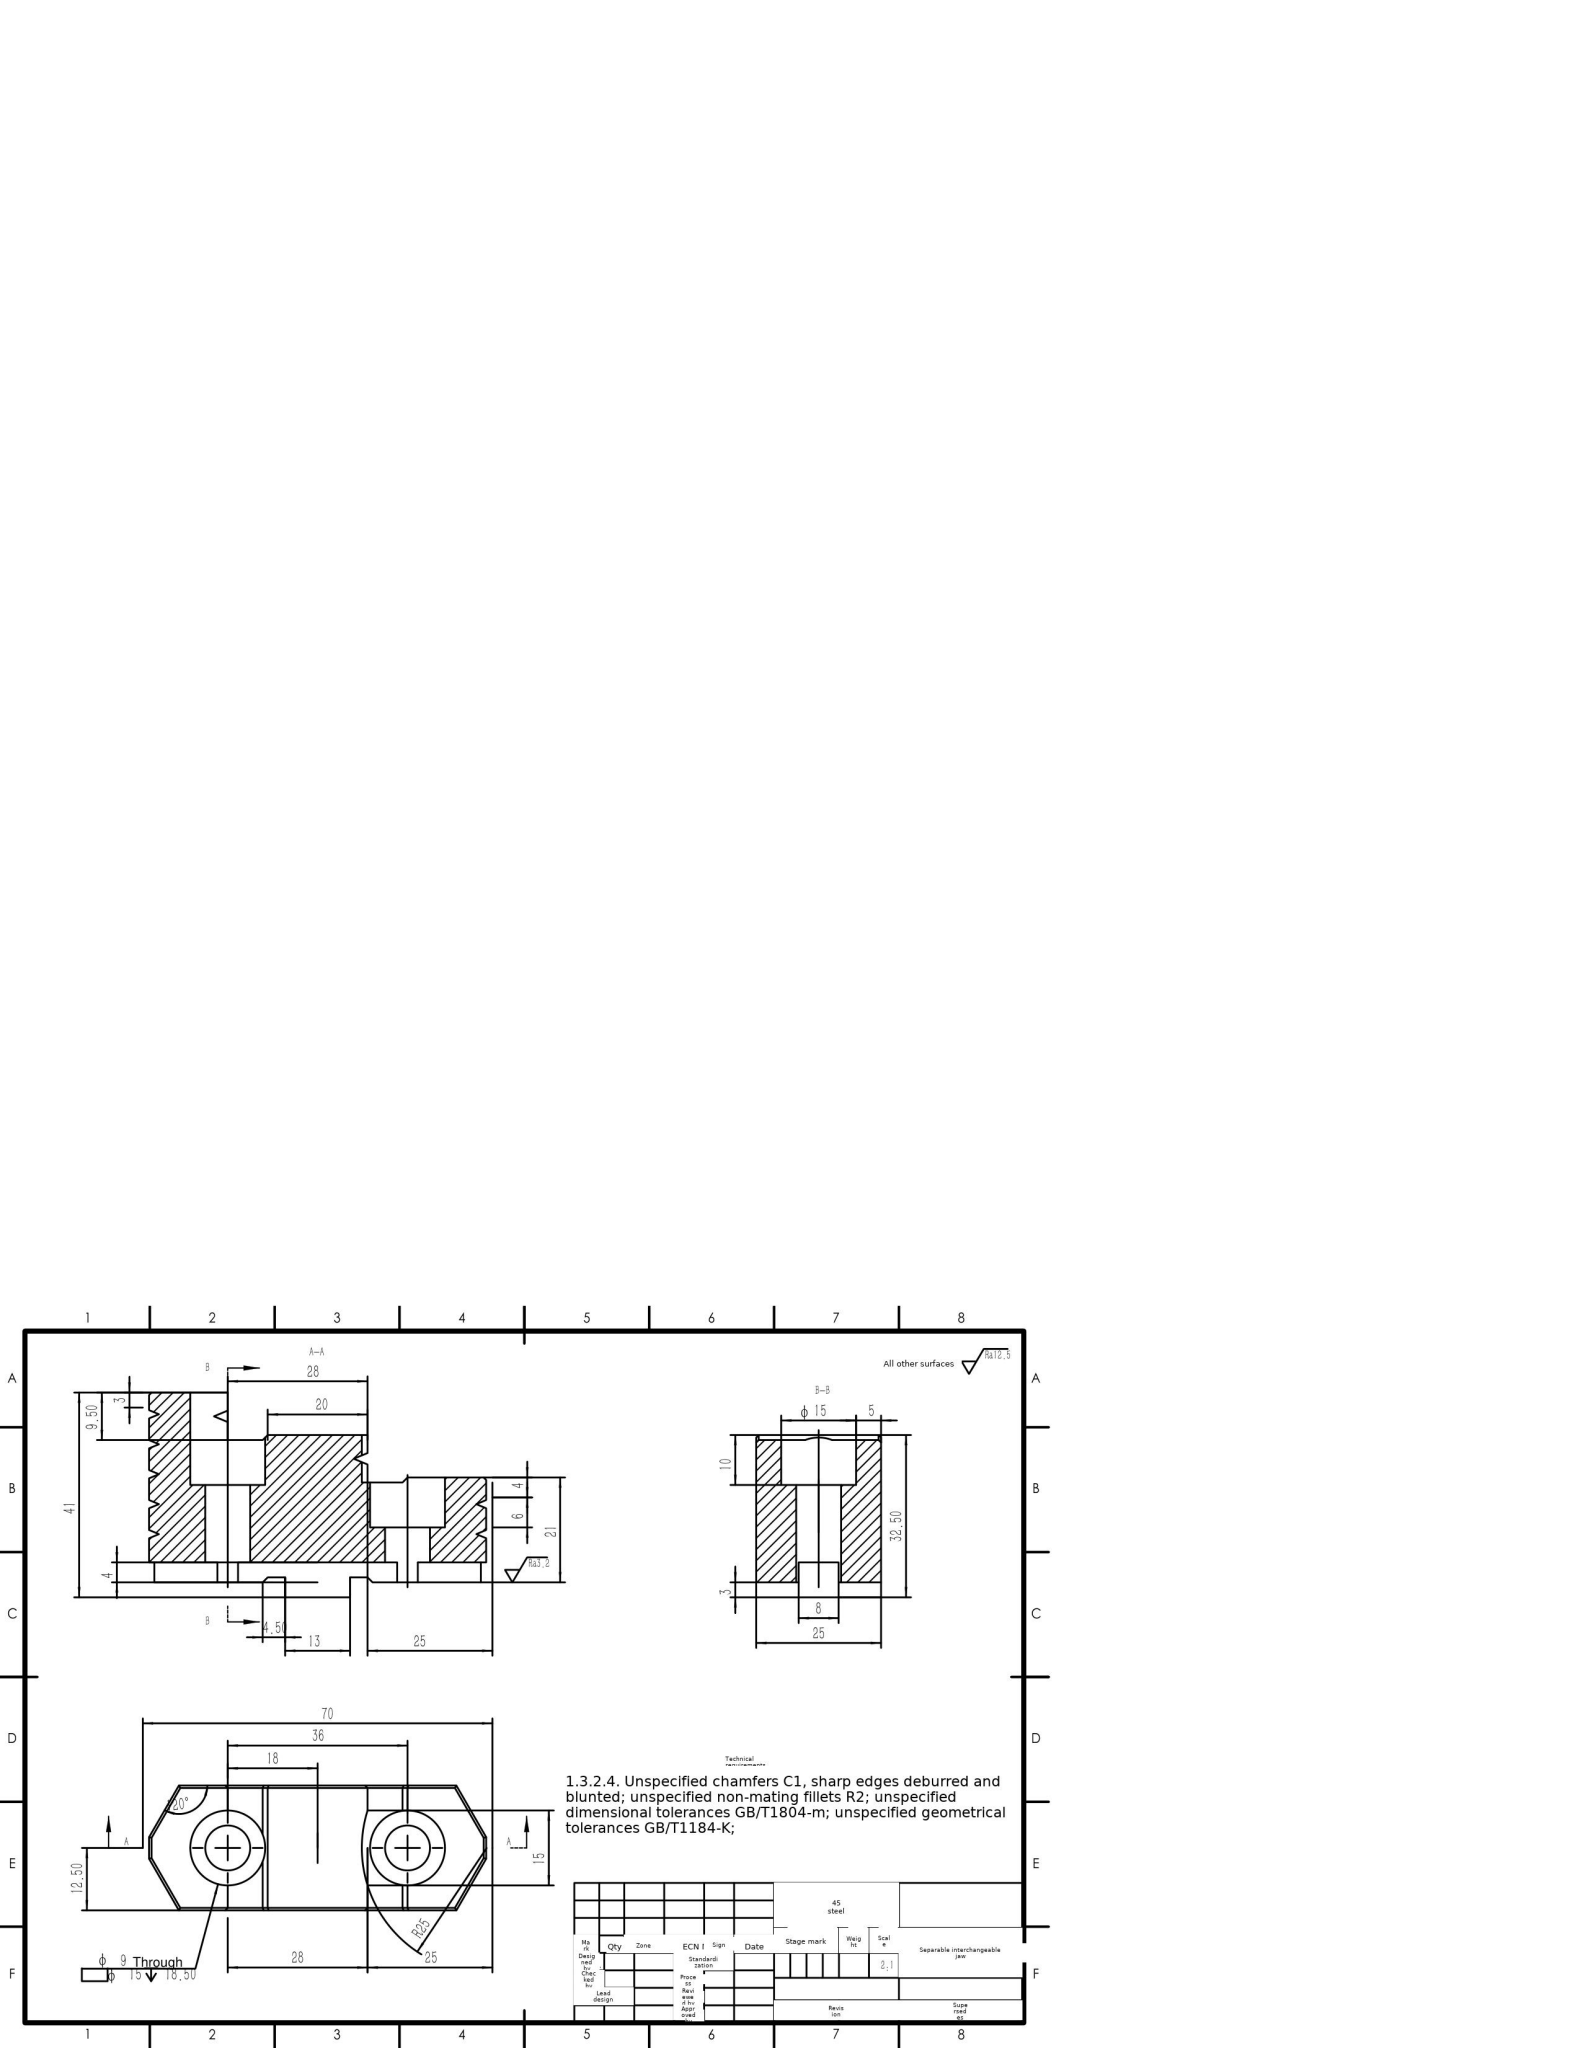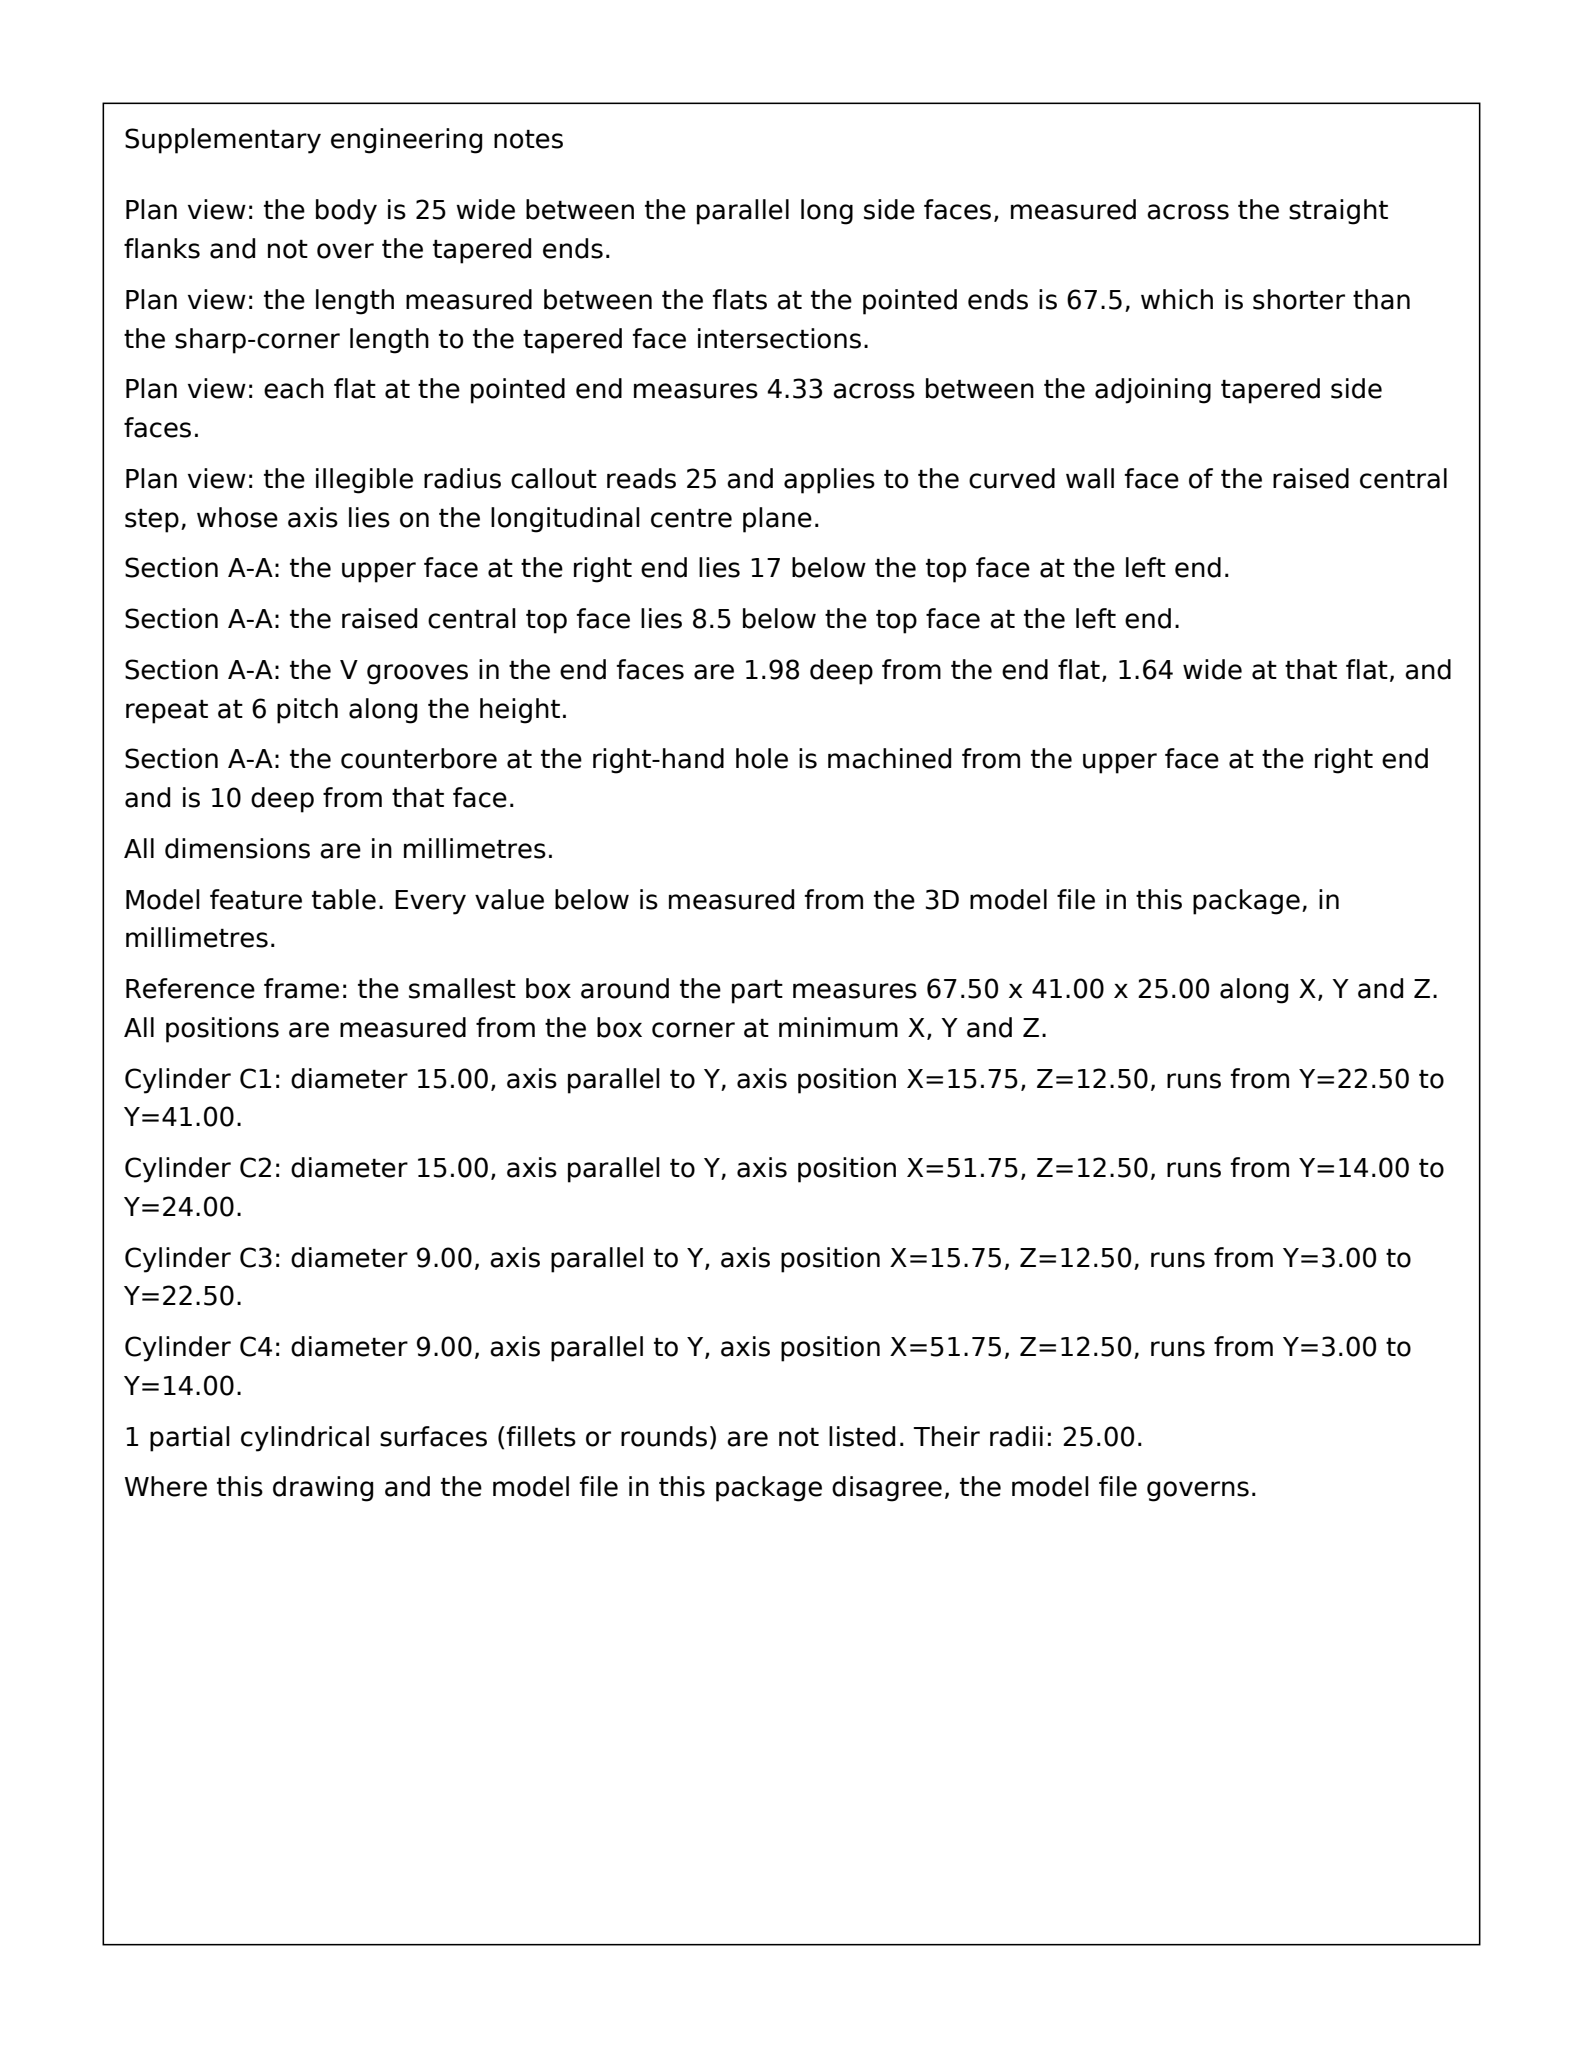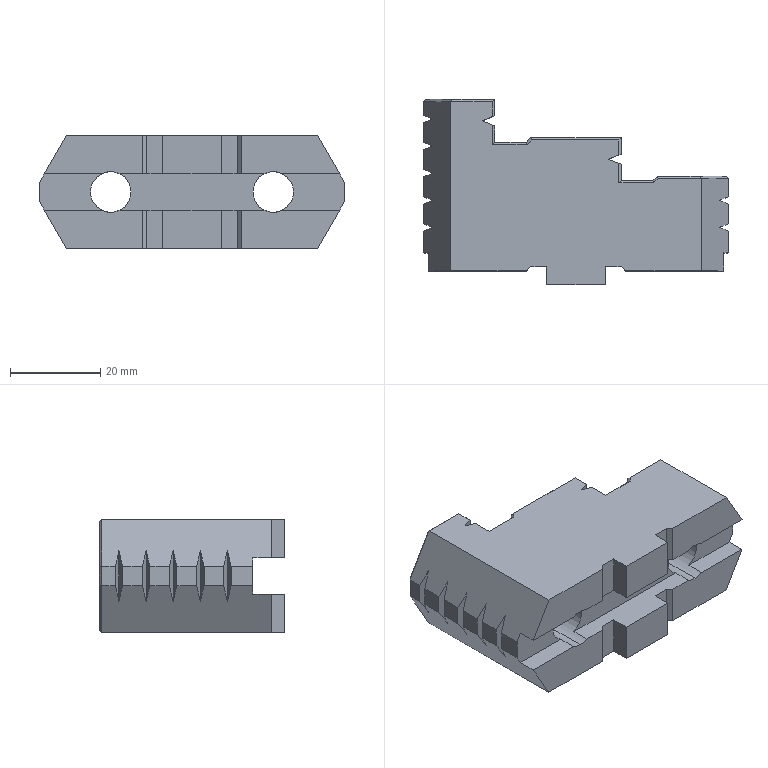Part | SolidWorks | mm | 1 solid | 119 faces | box 67.5 x 41 x 25 mm | volume 36580 mm3 | plane 109 | cylinder 10 | commonest cylinder face diameters 9 x4 15 x4 50 x2
Drawing notes:
2X Ø9 THRU, Ø15 C'BORE; HOLE CL 36 APART ON 12.50 Z CL | from the solid: Ø9 cyl, axis y, at x=15.75 and x=51.75, both z=12.5; spacing 51.75-15.75=36
RH HOLE (B-B): Ø15 C'BORE DP 10 | from the solid: [15.0,'y',[51.75,null,12.5],10.0] vs LH [15.0,'y',[15.75,null,12.5],9.5/18.5]
R25 ARC CTR 67.60 FROM LH END, ON 12.50 Z CL (BTM VIEW) | from the solid: cyl dia 50 (R25), axis y, pos [67.6,null,12.5], len 4.08, 2X
A-A BTM SLOT: 8 WIDE x 3 DEEP x 13 LG, 27.25 FROM LH END | from the solid: x-planes 27.25 & 40.25 (13 apart); z-planes 8.5 & 16.5 (8 wide, CL 12.5); y-plane 3.0
build123d program:
from build123d import *

# Parameters (mm, degrees)
BOSS_EXTRUDE1_DEPTH            = 38
CUT_EXTRUDE1_DEPTH             = 54.153
CUT_EXTRUDE1_DEPTH_BACK        = 54.153
CUT_EXTRUDE2_DEPTH             = 8.5
BOSS_EXTRUDE2_START            = 1
BOSS_EXTRUDE2_DEPTH            = 1
BOSS_EXTRUDE3_DEPTH            = 1
CUT_EXTRUDE3_DEPTH             = 54.153
CUT_EXTRUDE3_DEPTH_BACK        = 54.153
SKETCH6_W                      = 8
SKETCH6_H                      = 4
SKETCH7_W                      = 22
SKETCH7_H                      = 1
CUT_EXTRUDE4_DEPTH             = 58.393
SKETCH8_W                      = 13
SKETCH8_H                      = 8.5
BOSS_EXTRUDE4_DEPTH            = 4
DRAFT3_ANGLE                   = 45
DRAFT4_ANGLE                   = 45
DRAFT5_ANGLE                   = 45
DRAFT6_ANGLE                   = 45
DRAFT7_ANGLE                   = 45
DRAFT8_ANGLE                   = 45
CUT_EXTRUDE6_DEPTH             = 54.153
LPATTERN1_COUNT                = 5
LPATTERN1_PITCH                = 6
CUT_EXTRUDE7_DEPTH             = 54.153
LPATTERN2_COUNT                = 2
LPATTERN2_PITCH                = 6
CUT_EXTRUDE8_DEPTH             = 54.153
CUT_EXTRUDE8_DEPTH_BACK        = 54.153
CBORE_FOR_M8_SHCS2_D           = 9
CBORE_FOR_M8_SHCS2_CBORE_D     = 15
CBORE_FOR_M8_SHCS2_CBORE_DEPTH = 18.5
CBORE_FOR_M8_SHCS4_D           = 9
CBORE_FOR_M8_SHCS4_CBORE_D     = 15
CBORE_FOR_M8_SHCS4_CBORE_DEPTH = 10
CHAMFER1_SIZE                  = 2.5
CHAMFER1_EDGE_2_SIZE           = 2.5
CHAMFER1_EDGE_3_SIZE           = 2.5
CHAMFER1_EDGE_4_SIZE           = 2.5
CHAMFER1_EDGE_5_SIZE           = 2.5
CHAMFER1_EDGE_6_SIZE           = 2.5
CHAMFER1_EDGE_7_SIZE           = 2.5
CHAMFER1_EDGE_8_SIZE           = 2.5
CHAMFER1_EDGE_9_SIZE           = 2.5
CHAMFER2_SIZE                  = 0.5


with BuildPart() as part:
    # Sketch1 → Boss-Extrude1 (new body)
    with BuildSketch(Plane(origin=(0, 0, 0), x_dir=(1, 0, 0), z_dir=(0, 1, 0))):
        Polygon((27.783, -12.5), (-27.783, -12.5), (-35, 0), (-27.783, 12.5), (27.783, 12.5), (35, 0), align=None)
    extrude(amount=BOSS_EXTRUDE1_DEPTH)

    # Sketch2 → Cut-Extrude1 (cut, two sides: drawn at the far end of the back side and taken through both)
    with BuildSketch(Plane.XY.offset(-CUT_EXTRUDE1_DEPTH_BACK)):
        Polygon((-18, 38), (-18, 28.5), (10, 28.5), (10, 20), (35, 20), (35, 38), align=None)
    extrude(amount=CUT_EXTRUDE1_DEPTH + CUT_EXTRUDE1_DEPTH_BACK, mode=Mode.SUBTRACT)

    # Sketch3 → Cut-Extrude2 (cut)
    with BuildSketch(Plane(origin=(0, 28.5, 0), x_dir=(1, 0, 0), z_dir=(0, 1, 0))):
        with BuildLine():
            Line((10, 7.5), (10, -7.5))
            ThreePointArc((10, -7.5), (8.848, 0), (10, 7.5))
        make_face()
    extrude(amount=-CUT_EXTRUDE2_DEPTH, mode=Mode.SUBTRACT)

    # Sketch4 → Boss-Extrude2 (add)
    with BuildSketch(Plane(origin=(0, 28.5, 0), x_dir=(1, 0, 0), z_dir=(0, 1, 0)).offset(BOSS_EXTRUDE2_START)):
        with BuildLine():
            Line((-10, 12.5), (-10, -12.5))
            Line((-10, -12.5), (10, -12.5))
            Line((10, -12.5), (10, -7.5))
            ThreePointArc((10, -7.5), (8.848, 0), (10, 7.5))
            Line((10, 7.5), (10, 12.5))
            Line((10, 12.5), (-10, 12.5))
        make_face()
    extrude(amount=-BOSS_EXTRUDE2_DEPTH)

    # Sketch5 → Boss-Extrude3 (add)
    with BuildSketch(Plane(origin=(0, 20, 0), x_dir=(1, 0, 0), z_dir=(0, 1, 0))):
        Polygon((18, 12.5), (18, -12.5), (27.783, -12.5), (35, 0), (27.783, 12.5), align=None)
    extrude(amount=BOSS_EXTRUDE3_DEPTH)

    # Sketch6 → Cut-Extrude3 (cut, two sides: drawn at the far end of the back side and taken through both)
    with BuildSketch(Plane(origin=(0, 0, 0), x_dir=(0, 0, -1), z_dir=(1, 0, 0)).offset(-CUT_EXTRUDE3_DEPTH_BACK)):
        with Locations((0, 2)):
            Rectangle(SKETCH6_W, SKETCH6_H)
    extrude(amount=CUT_EXTRUDE3_DEPTH + CUT_EXTRUDE3_DEPTH_BACK, mode=Mode.SUBTRACT)

    # Sketch7 → Cut-Extrude4 (cut, through all)
    with BuildSketch(Plane.XY.offset(12.5)):
        with Locations((0, 0.5)):
            Rectangle(SKETCH7_W, SKETCH7_H)
    extrude(amount=-CUT_EXTRUDE4_DEPTH, mode=Mode.SUBTRACT)

    # Sketch8 → Boss-Extrude4 (add)
    with BuildSketch(Plane.XZ.offset(-1)):
        with Locations((0, 8.25)):
            Rectangle(SKETCH8_W, SKETCH8_H)
        with Locations((0, -8.25)):
            Rectangle(SKETCH8_W, SKETCH8_H)
    extrude(amount=BOSS_EXTRUDE4_DEPTH)

    # Draft3
    draft3_faces = [part.faces().sort_by_distance(p)[0] for p in [
        (-11, 0.5, -8.25),
    ]]
    draft(draft3_faces, Plane(origin=(0, 0, 0), x_dir=(0, 0, -1), z_dir=(0, -1, 0)), DRAFT3_ANGLE)

    # Draft4
    draft4_faces = [part.faces().sort_by_distance(p)[0] for p in [
        (-11, 0.5, 8.25),
    ]]
    draft(draft4_faces, Plane(origin=(0, 0, 0), x_dir=(0, 0, -1), z_dir=(0, -1, 0)), DRAFT4_ANGLE)

    # Draft5
    draft5_faces = [part.faces().sort_by_distance(p)[0] for p in [
        (11, 0.5, -8.25),
    ]]
    draft(draft5_faces, Plane(origin=(0, 0, 0), x_dir=(0, 0, -1), z_dir=(0, -1, 0)), DRAFT5_ANGLE)

    # Draft6
    draft6_faces = [part.faces().sort_by_distance(p)[0] for p in [
        (11, 0.5, 8.25),
    ]]
    draft(draft6_faces, Plane(origin=(0, 0, 0), x_dir=(0, 0, -1), z_dir=(0, -1, 0)), DRAFT6_ANGLE)

    # Draft7
    draft7_faces = [part.faces().sort_by_distance(p)[0] for p in [
        (-10, 29, 0),
    ]]
    draft(draft7_faces, Plane(origin=(33.848, 29.5, 0), x_dir=(0, 0, 1), z_dir=(0, 1, 0)), DRAFT7_ANGLE)

    # Draft8
    draft8_faces = [part.faces().sort_by_distance(p)[0] for p in [
        (18, 20.5, 0),
    ]]
    draft(draft8_faces, Plane.ZX.offset(21), DRAFT8_ANGLE)

    # Sketch9 → Cut-Extrude6 (cut, symmetric)
    with BuildSketch(Plane.XY):
        Polygon((-35, 35), (-31.766, 33.661), (-35, 32.321), align=None)
    cut_extrude6 = extrude(amount=CUT_EXTRUDE6_DEPTH, both=True, mode=Mode.SUBTRACT)

    # LPattern1: Cut-Extrude6 ×5
    with Locations(*[(0, -i * LPATTERN1_PITCH, 0) for i in range(1, LPATTERN1_COUNT)]):
        add(cut_extrude6, mode=Mode.SUBTRACT)

    # Sketch10 → Cut-Extrude7 (cut, symmetric)
    with BuildSketch(Plane.XY):
        Polygon((35, 17), (31.766, 15.661), (35, 14.321), align=None)
    cut_extrude7 = extrude(amount=CUT_EXTRUDE7_DEPTH, both=True, mode=Mode.SUBTRACT)

    # LPattern2: Cut-Extrude7 ×2
    with Locations(*[(0, -i * LPATTERN2_PITCH, 0) for i in range(1, LPATTERN2_COUNT)]):
        add(cut_extrude7, mode=Mode.SUBTRACT)

    # Sketch11 → Cut-Extrude8 (cut, two sides: drawn at the far end of the back side and taken through both)
    with BuildSketch(Plane.XY.offset(-CUT_EXTRUDE8_DEPTH_BACK)):
        Polygon((-18, 34.398), (-18, 32.102), (-20.772, 33.25), align=None)
        Polygon((7.228, 24.75), (10, 25.898), (10, 23.602), align=None)
    extrude(amount=CUT_EXTRUDE8_DEPTH + CUT_EXTRUDE8_DEPTH_BACK, mode=Mode.SUBTRACT)

    # CBORE for M8 SHCS2 (through all)
    with Locations(Plane(origin=(-18, 38, 0), x_dir=(0, 0, 1), z_dir=(0, 1, 0))):
        with Locations((0, 0)):
            CounterBoreHole(CBORE_FOR_M8_SHCS2_D / 2, CBORE_FOR_M8_SHCS2_CBORE_D / 2, CBORE_FOR_M8_SHCS2_CBORE_DEPTH)

    # CBORE for M8 SHCS4 (through all)
    with Locations(Plane(origin=(18, 21, 0), x_dir=(0, 0, 1), z_dir=(0, 1, 0))):
        with Locations((0, 0)):
            CounterBoreHole(CBORE_FOR_M8_SHCS4_D / 2, CBORE_FOR_M8_SHCS4_CBORE_D / 2, CBORE_FOR_M8_SHCS4_CBORE_DEPTH)

    # Chamfer1
    chamfer1_edges = [part.edges().sort_by_distance(p)[0] for p in [
        (-35, 36.5, 0),
    ]]
    chamfer(chamfer1_edges, length=CHAMFER1_SIZE)

    # Chamfer1 edge 2
    chamfer1_edge_2_edges = [part.edges().sort_by_distance(p)[0] for p in [
        (-35, 30.661, 0),
    ]]
    chamfer(chamfer1_edge_2_edges, length=CHAMFER1_EDGE_2_SIZE)

    # Chamfer1 edge 3
    chamfer1_edge_3_edges = [part.edges().sort_by_distance(p)[0] for p in [
        (-35, 24.661, 0),
    ]]
    chamfer(chamfer1_edge_3_edges, length=CHAMFER1_EDGE_3_SIZE)

    # Chamfer1 edge 4
    chamfer1_edge_4_edges = [part.edges().sort_by_distance(p)[0] for p in [
        (-35, 18.661, 0),
    ]]
    chamfer(chamfer1_edge_4_edges, length=CHAMFER1_EDGE_4_SIZE)

    # Chamfer1 edge 5
    chamfer1_edge_5_edges = [part.edges().sort_by_distance(p)[0] for p in [
        (-35, 12.661, 0),
    ]]
    chamfer(chamfer1_edge_5_edges, length=CHAMFER1_EDGE_5_SIZE)

    # Chamfer1 edge 6
    chamfer1_edge_6_edges = [part.edges().sort_by_distance(p)[0] for p in [
        (-35, 6.161, 0),
    ]]
    chamfer(chamfer1_edge_6_edges, length=CHAMFER1_EDGE_6_SIZE)

    # Chamfer1 edge 7
    chamfer1_edge_7_edges = [part.edges().sort_by_distance(p)[0] for p in [
        (35, 19, 0),
    ]]
    chamfer(chamfer1_edge_7_edges, length=CHAMFER1_EDGE_7_SIZE)

    # Chamfer1 edge 8
    chamfer1_edge_8_edges = [part.edges().sort_by_distance(p)[0] for p in [
        (35, 12.661, 0),
    ]]
    chamfer(chamfer1_edge_8_edges, length=CHAMFER1_EDGE_8_SIZE)

    # Chamfer1 edge 9
    chamfer1_edge_9_edges = [part.edges().sort_by_distance(p)[0] for p in [
        (35, 6.161, 0),
    ]]
    chamfer(chamfer1_edge_9_edges, length=CHAMFER1_EDGE_9_SIZE)

    # Chamfer2
    chamfer2_edges = [part.edges().sort_by_distance(p)[0] for p in [
        (-22.892, 38, -12.5),
        (-30.767, 38, -7.333),
        (13.5, 20, -12.5),
        (13.5, 20, 12.5),
        (-18, 36.199, 12.5),
        (-14.5, 28.5, 12.5),
        (10, 27.699, 12.5),
        (10, 27.699, -12.5),
        (-14.5, 28.5, -12.5),
        (-18, 36.199, -12.5),
        (-18, 30.301, -12.5),
        (-18, 30.301, 12.5),
        (10, 21.801, -12.5),
        (10, 21.801, 12.5),
        (30.767, 21, -7.333),
        (33.75, 21, 0),
        (-30.767, 38, 7.333),
        (-33.75, 38, 0),
        (-10.5, 29, 12.5),
        (-10.5, 29, -12.5),
        (0, 29.5, 12.5),
        (0, 29.5, -12.5),
        (17.5, 20.5, -12.5),
        (17.5, 20.5, 12.5),
        (30.767, 21, 7.333),
        (22.892, 21, -12.5),
        (22.892, 21, 12.5),
        (-22.892, 38, 12.5),
    ]]
    chamfer(chamfer2_edges, length=CHAMFER2_SIZE)


solid = part.part